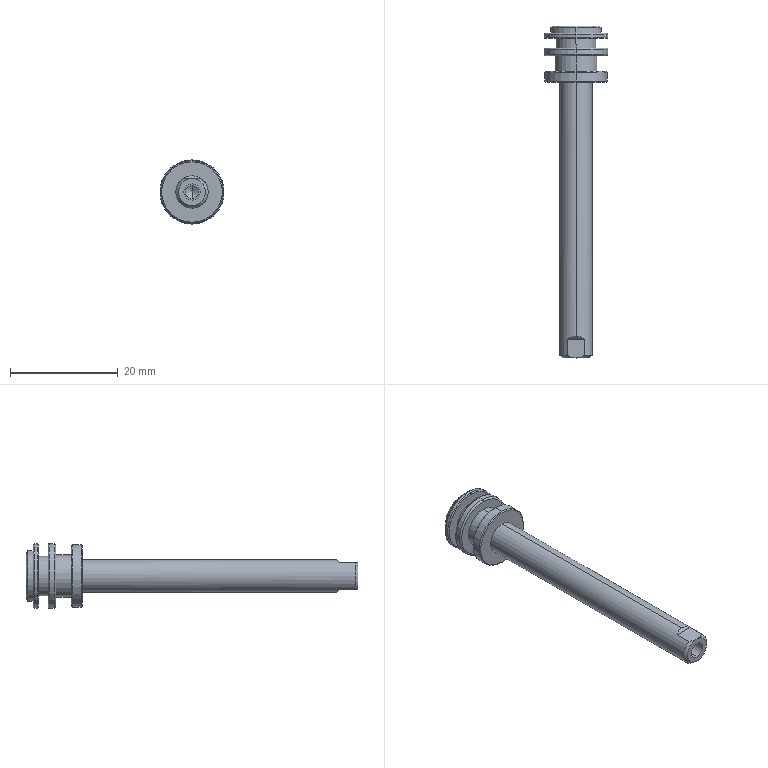Component | SolidWorks | TC_L_12x30_S_0-1_TC_L_12x30_30r-1 | 1 solid | 49 faces | box 11.9 x 61.5 x 11.9 mm | volume 2154 mm3 | cylinder 18 | plane 13 | cone 10 | torus 8 | commonest cylinder face diameters 11.9 x4 2.459 x2 3 x2 9.4 x2 7.4 x2 7.8 x2 11.6 x2 6 x2
build123d program:
from build123d import *

# Parameters (mm, degrees)
CUT_EXTRUDE1_DEPTH      = 10
CUT_EXTRUDE1_DEPTH_BACK = 10
SKETCH1_R               = 1.5
M3_THREAD_MAJOR_DEPTH   = 6


with BuildPart() as part:
    # Sketch1_2 → Revolve1 (revolve)
    with BuildSketch(Plane.XY, mode=Mode.PRIVATE) as revolve1_sk:
        with BuildLine():
            Line((0, 0), (0, 2.5))
            Line((0, 2.5), (0.5, 3))
            Line((0.5, 3), (51.1, 3))
            Line((51.1, 3), (51.1, 5.6))
            Line((51.1, 5.6), (51.3, 5.8))
            Line((51.3, 5.8), (52.9, 5.8))
            Line((52.9, 5.8), (53.1, 5.6))
            Line((53.1, 5.6), (53.1, 3.9))
            Line((53.1, 3.9), (56, 3.9))
            Line((56, 3.9), (56, 5.65))
            ThreePointArc((56, 5.65), (56.088, 5.862), (56.3, 5.95))
            Line((56.3, 5.95), (57.2, 5.95))
            ThreePointArc((57.2, 5.95), (57.341, 5.891), (57.4, 5.75))
            Line((57.4, 5.75), (57.4, 3.7))
            Line((57.4, 3.7), (59.2, 3.7))
            Line((59.2, 3.7), (59.2, 5.75))
            ThreePointArc((59.2, 5.75), (59.259, 5.891), (59.4, 5.95))
            Line((59.4, 5.95), (59.9, 5.95))
            ThreePointArc((59.9, 5.95), (60.112, 5.862), (60.2, 5.65))
            Line((60.2, 5.65), (60.2, 4.7))
            Line((60.2, 4.7), (61.2, 4.7))
            Line((61.2, 4.7), (61.5, 4.4))
            Line((61.5, 4.4), (61.5, 0))
            Line((61.5, 0), (0, 0))
        make_face()
    revolve(revolve1_sk.sketch.rotate(Axis((61.5, 0, 0), (-1, 0, 0)), 270), axis=Axis((61.5, 0, 0), (-1, 0, 0)))

    # Sketch2 → Cut-Extrude1 (cut, two sides: drawn at the far end of the back side and taken through both)
    with BuildSketch(Plane(origin=(0, 0, 0), x_dir=(1, 0, 0), z_dir=(0, 1, 0)).offset(-CUT_EXTRUDE1_DEPTH_BACK)):
        Polygon((-5, 9.571), (-5, -9.571), (10.571, -9.571), (3.5, -2.5), (0, -2.5), (0, 2.5), (3.5, 2.5), (10.571, 9.571), align=None)
    extrude(amount=CUT_EXTRUDE1_DEPTH + CUT_EXTRUDE1_DEPTH_BACK, mode=Mode.SUBTRACT)

    # Sketch3 → Cut-Revolve1 (revolve, cut)
    with BuildSketch(Plane.XY, mode=Mode.PRIVATE) as cut_revolve1_sk:
        Polygon((0, 0), (0, 1.5), (0.2705, 1.23), (9.6, 1.23), (10.31, 0), align=None)
    revolve(cut_revolve1_sk.sketch.rotate(Axis((10.31, 0, 0), (-1, 0, 0)), 270), axis=Axis((10.31, 0, 0), (-1, 0, 0)), mode=Mode.SUBTRACT)

    # Sketch1 → M3_Thread_Major (cut)
    with BuildSketch(Plane.ZY):
        Circle(SKETCH1_R)
    extrude(amount=-M3_THREAD_MAJOR_DEPTH, mode=Mode.SUBTRACT)


solid = part.part

# Placed as in the assembly
solid = solid.moved(Location((-42, 169.3, 57), (0, 0, 90)))